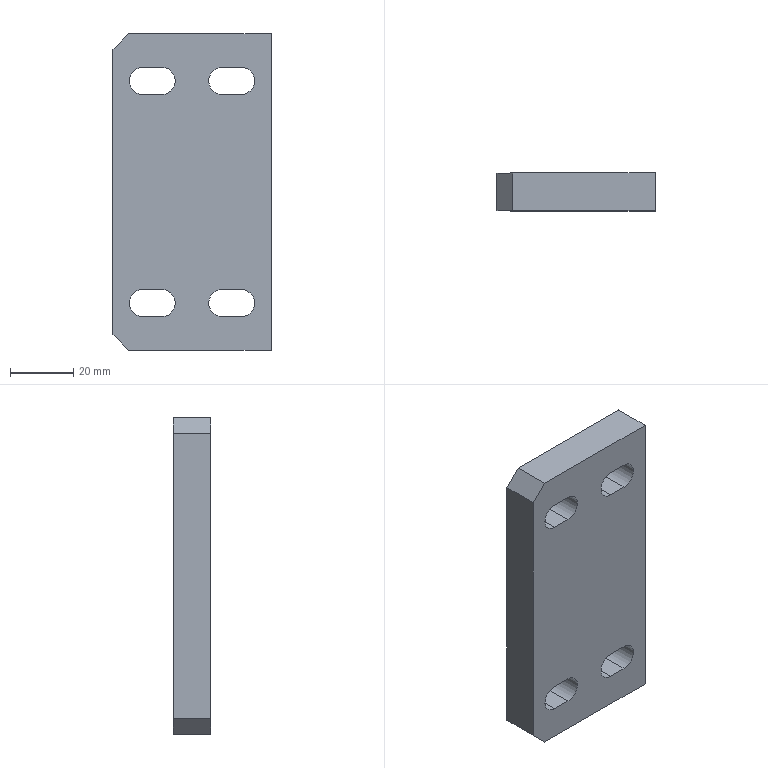Component | SolidWorks | ChainPartMotorMountFootPlate-1 | 1 solid | 36 faces | box 49.8 x 11.8 x 99.8 mm | volume 52911 mm3 | cylinder 16 | plane 16 | cone 4 | commonest cylinder face diameters 8.5 x12 4.2 x4
build123d program:
from build123d import *

# Parameters (mm, degrees)
SKETCH6_W             = 49.8
SKETCH6_H             = 11.8
BOSS_EXTRUDE2_DEPTH   = 49.9
M5_TAPPED_HOLE1_D     = 4.2
M5_TAPPED_HOLE1_DEPTH = 12.4
M5_TAPPED_HOLE1_TIP   = 1.262
CUT_EXTRUDE1_DEPTH    = 58.002
CHAMFER1_SIZE         = 5


with BuildPart() as part:
    # Sketch6 → Boss-Extrude2 (new, symmetric)
    with BuildSketch(Plane.ZY):
        Rectangle(SKETCH6_W, SKETCH6_H)
    extrude(amount=BOSS_EXTRUDE2_DEPTH, both=True)

    # M5 Tapped Hole1
    with Locations(Plane(origin=(0, 0, -24.9), x_dir=(-1, 0, 0), z_dir=(0, 0, -1))):
        with Locations((-25, 0), (25, 0)):
            Hole(M5_TAPPED_HOLE1_D / 2, depth=M5_TAPPED_HOLE1_DEPTH)
            with Locations((0, 0, -(M5_TAPPED_HOLE1_DEPTH + M5_TAPPED_HOLE1_TIP / 2))):  # 118° drill point
                Cone(0, M5_TAPPED_HOLE1_D / 2, M5_TAPPED_HOLE1_TIP, mode=Mode.SUBTRACT)

    # Sketch11 → Cut-Extrude1 (cut, through all)
    with BuildSketch(Plane(origin=(0, 5.9, 0), x_dir=(1, 0, 0), z_dir=(0, 1, 0))):
        with BuildLine():
            Line((-30.75, 15.5), (-30.75, 9.5))
            ThreePointArc((-30.75, 9.5), (-35, 5.25), (-39.25, 9.5))
            Line((-39.25, 9.5), (-39.25, 15.5))
            ThreePointArc((-39.25, 15.5), (-35, 19.75), (-30.75, 15.5))
        make_face()
        with BuildLine():
            Line((-30.75, -9.5), (-30.75, -15.5))
            ThreePointArc((-30.75, -15.5), (-35, -19.75), (-39.25, -15.5))
            Line((-39.25, -15.5), (-39.25, -9.5))
            ThreePointArc((-39.25, -9.5), (-35, -5.25), (-30.75, -9.5))
        make_face()
        with BuildLine():
            Line((39.25, 15.5), (39.25, 9.5))
            ThreePointArc((39.25, 9.5), (35, 5.25), (30.75, 9.5))
            Line((30.75, 9.5), (30.75, 15.5))
            ThreePointArc((30.75, 15.5), (35, 19.75), (39.25, 15.5))
        make_face()
        with BuildLine():
            Line((39.25, -9.5), (39.25, -15.5))
            ThreePointArc((39.25, -15.5), (35, -19.75), (30.75, -15.5))
            Line((30.75, -15.5), (30.75, -9.5))
            ThreePointArc((30.75, -9.5), (35, -5.25), (39.25, -9.5))
        make_face()
    extrude(amount=-CUT_EXTRUDE1_DEPTH, mode=Mode.SUBTRACT)

    # Chamfer1
    chamfer1_edges = [part.edges().sort_by_distance(p)[0] for p in [
        (49.9, 0, 24.9),
        (-49.9, 0, 24.9),
    ]]
    chamfer(chamfer1_edges, length=CHAMFER1_SIZE)


solid = part.part

# Placed as in the assembly
solid = solid.moved(Location((203.937, 69.037, -35.304), (0, -90, 0)))